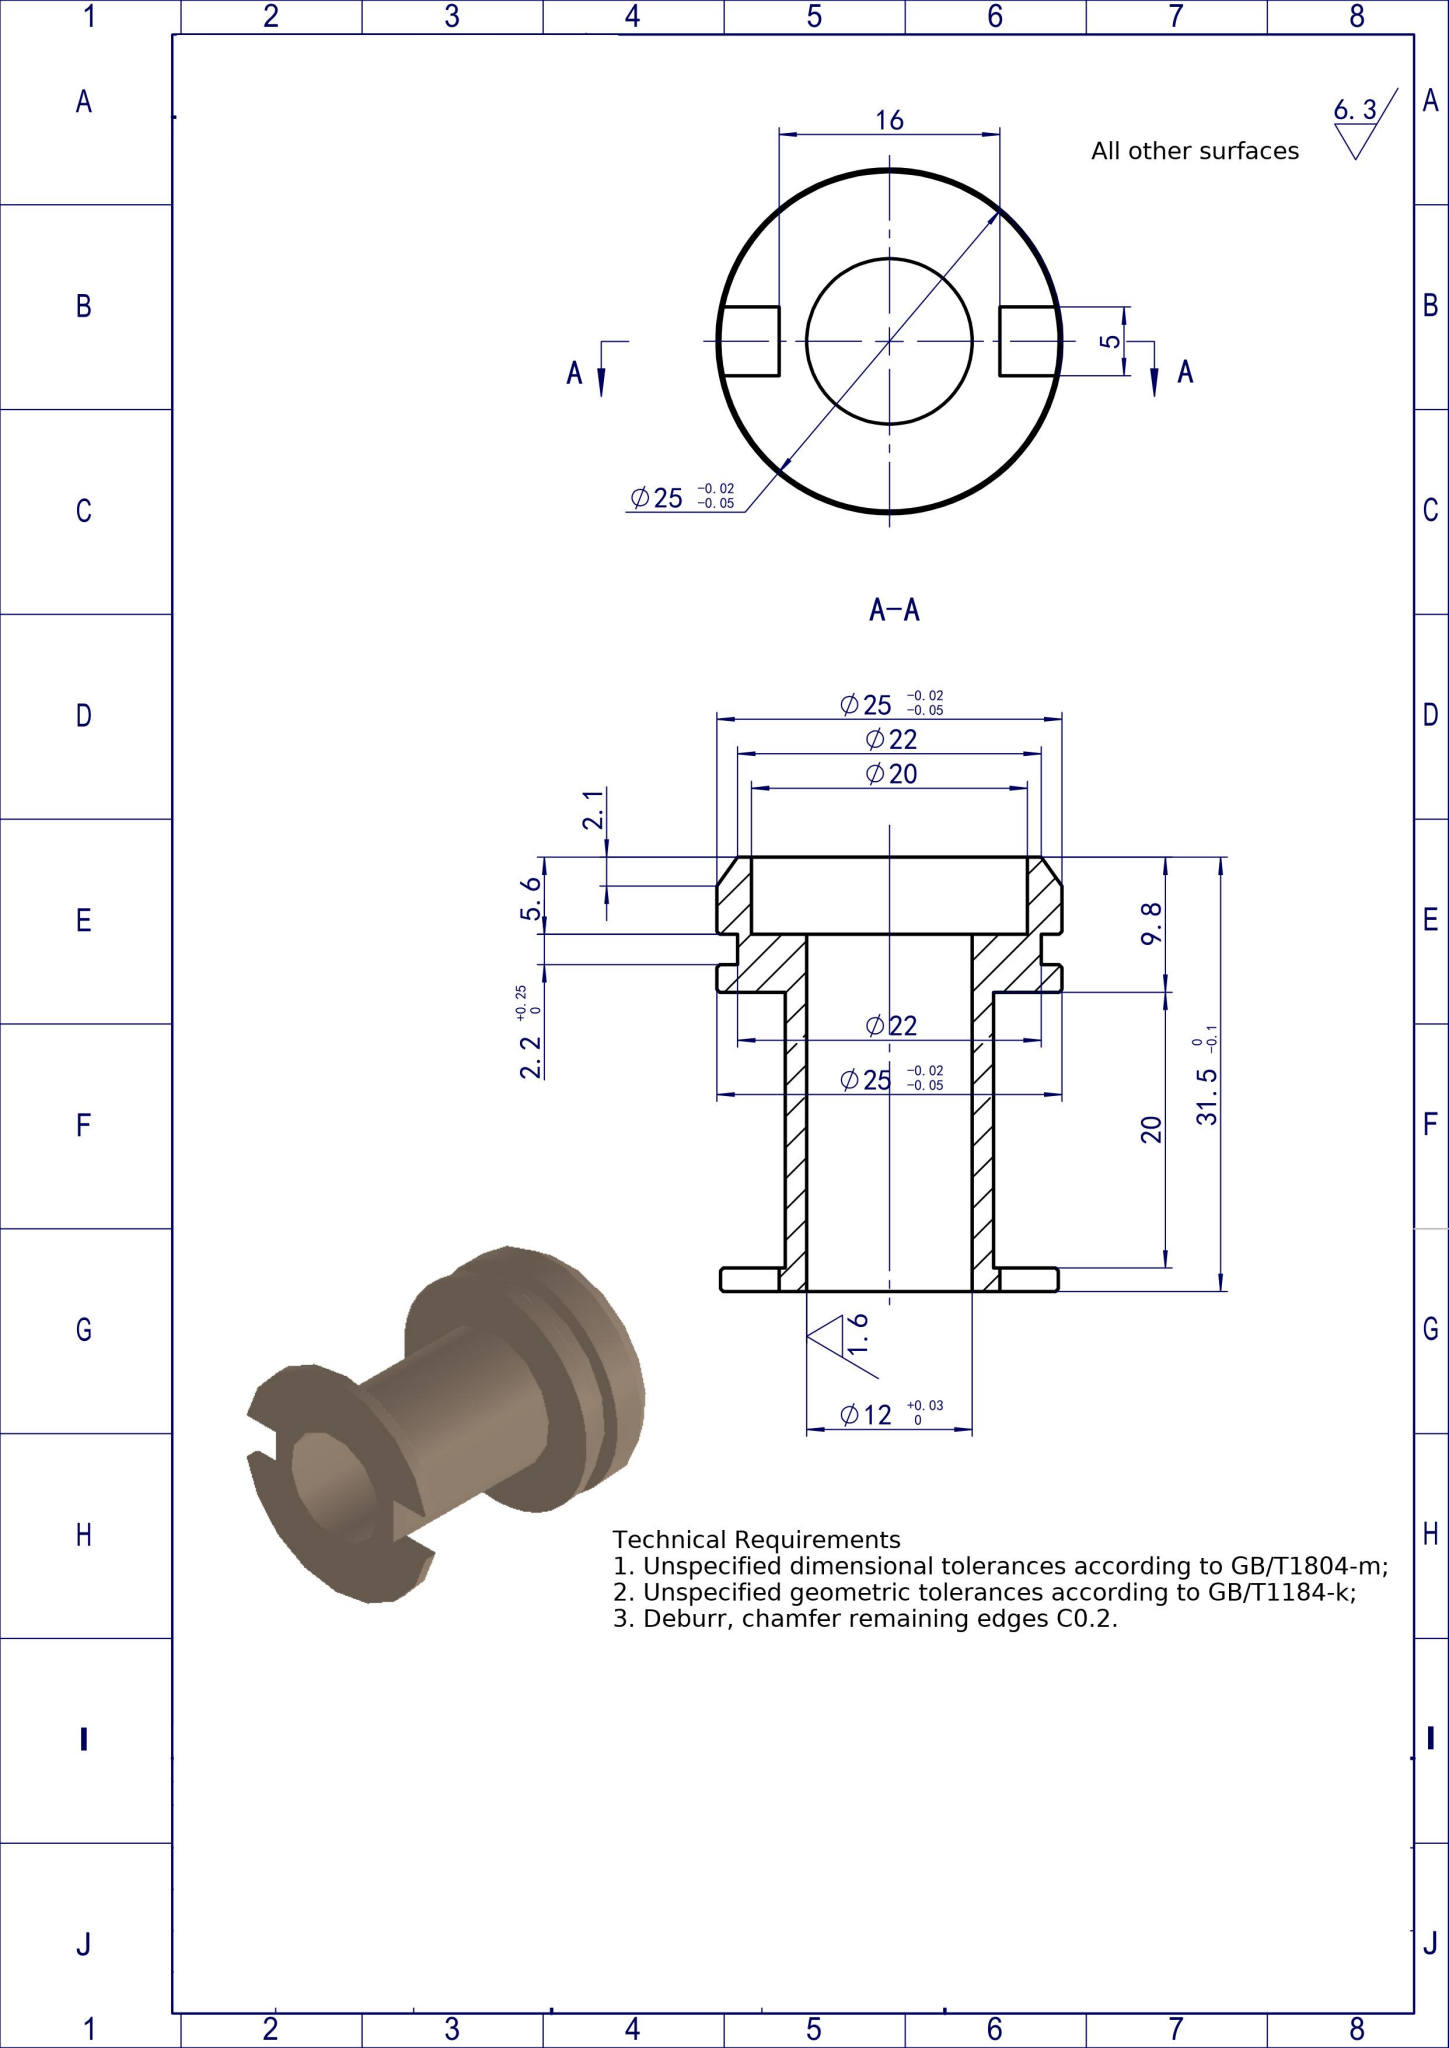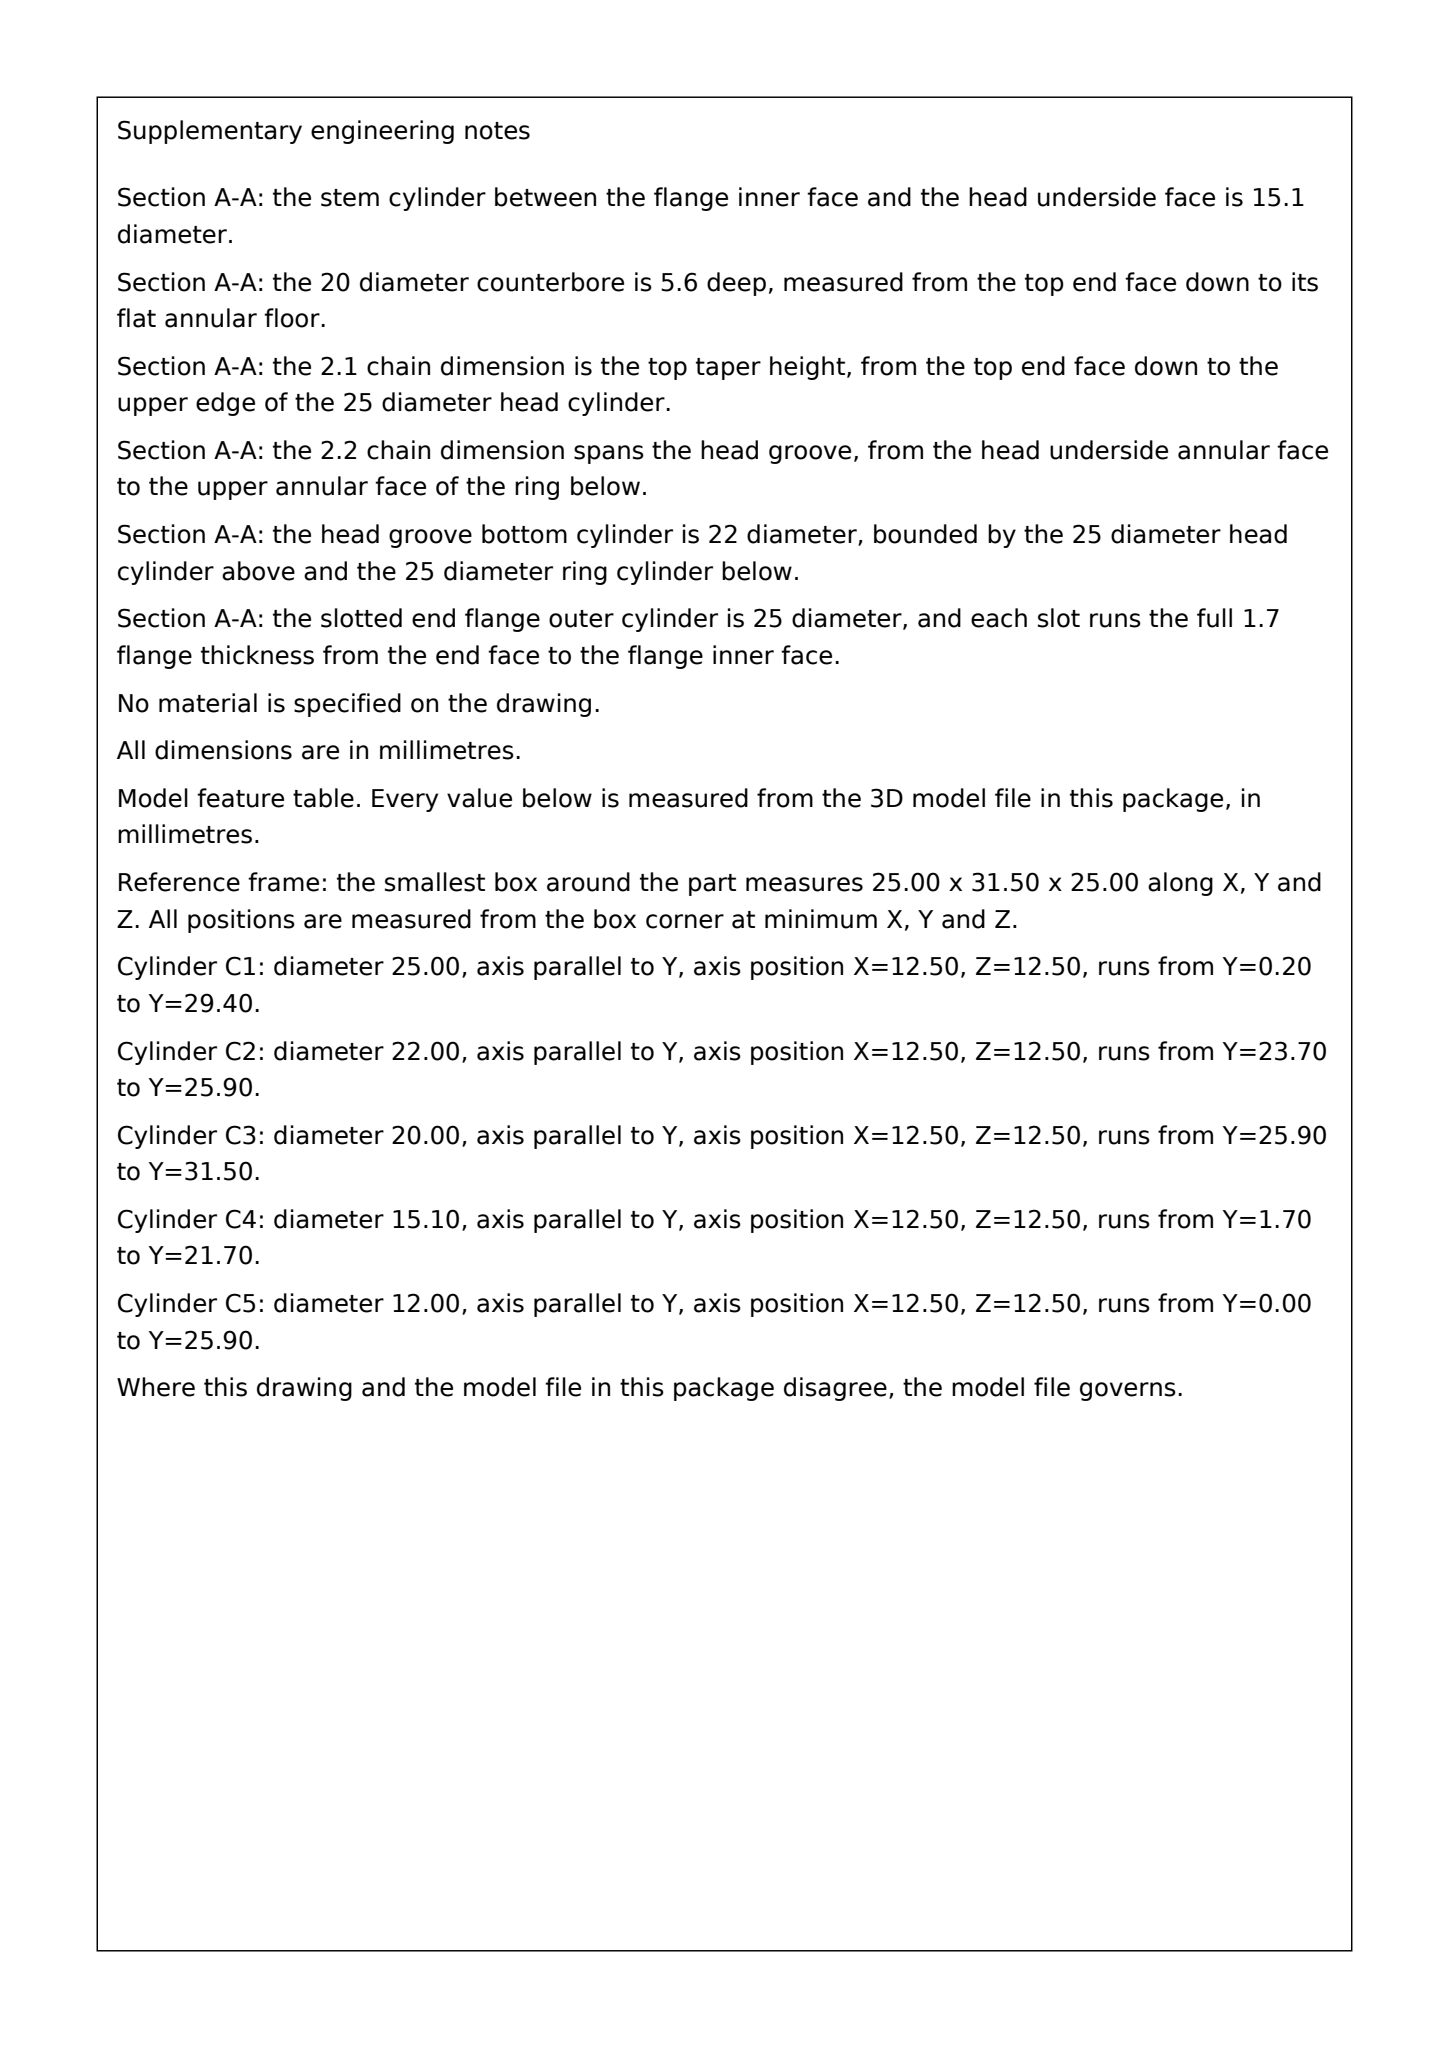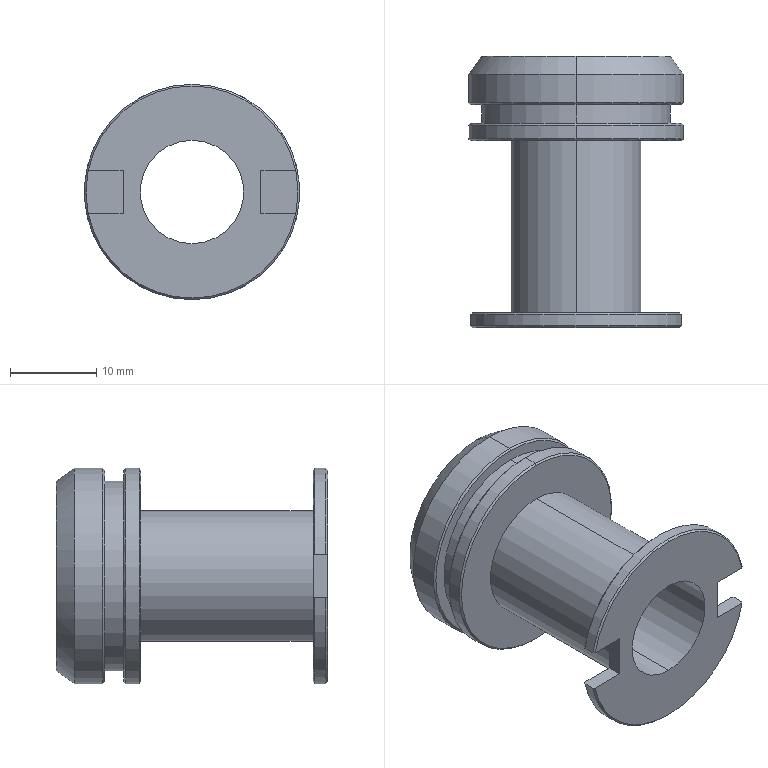Part | SolidWorks | mm | 1 solid | 42 faces | box 25 x 31.5 x 25 mm | volume 4093 mm3 | cylinder 15 | cone 14 | plane 13 | commonest cylinder face diameters 25 x7 20 x2 22 x2 15.1 x2 12 x2
Drawing notes:
2 SLOTS 5 WIDE x 16 ACROSS FLATS DP 5.6 FROM Ø25 FLANGE FACE | from the solid: Slot flats at x=4.5 & 20.5 (16 apart), walls z=10.0/15.0 (5 wide); slot floors = planes y=25.9 (2 off), i.e. 31.5-25.9=5.6 below flange face y=31.5
EXT GROOVE ON Ø25 FLANGE OD: 2.1 WIDE x Ø22 MINOR DIA | from the solid: Only sub-Ø25 external cyl in flange zone: Ø22 about axis y at [12.5,12.5], L=2.2, between Ø25 bands; drawing width 2.1
Ø25 BANDS 1.6 & 1.3 WIDE BTWN 5.6 AND 9.8 FROM FLANGE FACE | from the solid: Ø25 cyls L=1.6 and L=1.3 lie between planes y=21.7 and y=25.9, i.e. 9.8 and 5.6 below flange face y=31.5
FLANGE UNDERSIDE UNDERCUT: 71.1° INCL CONE FROM Ø25 AT 5.6 | from the solid: cones[71.1, ref_dia 25.0] x2 at flange underside, starts at Ø25 at plane y=25.9 = 5.6 from flange face y=31.5
Ø25 LANDS 3.3 & 1.6 WIDE: 2.1-5.4 AND 8.0-9.6 FROM TOP FACE | from the solid: Ø25 cyls L=3.3 (y 26.1-29.4) & L=1.6 (y 21.9-23.5); top face y=31.5; y-planes 21.7/23.7/25.9/31.5
RELIEF BTWN Ø25 LANDS: Ø22 x 2.2 WIDE; CHAMFER RUNOUT Ø24.6 | from the solid: Ø22 cyl L=2.2 between y-planes 23.7 and 25.9; 90° cones ref dia 24.6/25.0
Ø22 EXT GROOVE 2.2 WIDE, 5.6 FROM TOP FACE TO NEAR SIDE | from the solid: Ø22 cyl L=2.2 spans y 23.7-25.9; top face y=31.5 -> 31.5-25.9=5.6
ALL Ø25 LAND END EDGES C0.2 x 45° (TO Ø24.6) | from the solid: 90° included cones, ref dia 25.0 -> 24.6: 0.2 radial = 0.2 axial
build123d program:
from build123d import *

# Parameters (mm, degrees)
CHAMFER1_SIZE      = 0.2
CUT_EXTRUDE1_REACH = 38.121
SKETCH2_W          = 10
SKETCH2_H          = 5


with BuildPart() as part:
    # Sketch1 → Revolve1 (revolve)
    with BuildSketch(Plane.XY, mode=Mode.PRIVATE) as revolve1_sk:
        Polygon((6, 0), (12.5, 0), (12.5, 1.7), (7.55, 1.7), (7.55, 21.7), (12.5, 21.7), (12.5, 23.7), (11, 23.7), (11, 25.9), (12.5, 25.9), (12.5, 29.4), (11, 31.5), (10, 31.5), (10, 25.9), (6, 25.9), align=None)
    revolve(revolve1_sk.sketch.rotate(Axis((0, 0, 0), (0, 1, 0)), 90), axis=Axis((0, 0, 0), (0, 1, 0)))

    # Chamfer1
    chamfer1_edges = [part.edges().sort_by_distance(p)[0] for p in [
        (0, 25.9, 12.5),
        (0, 23.7, 12.5),
        (0, 21.7, 12.5),
        (0, 1.7, 12.5),
        (0, 0, 12.5),
    ]]
    chamfer(chamfer1_edges, length=CHAMFER1_SIZE)

    # Cut-Extrude1: up to this face of the body (flat: up to its plane)
    cut_extrude1_end = Plane(part.part.faces().sort_by_distance((0, 1.7, 11.952))[0])
    # Sketch2 → Cut-Extrude1 (cut, up to the picked face)
    with BuildSketch(Plane(origin=(0, 0, 0), x_dir=(-1, 0, 0), z_dir=(0, -1, 0)), mode=Mode.PRIVATE) as cut_extrude1_sk1:
        with Locations((-13, 0)):
            Rectangle(SKETCH2_W, SKETCH2_H)
    cut_extrude1_tool1 = split(extrude(cut_extrude1_sk1.sketch, amount=-CUT_EXTRUDE1_REACH, mode=Mode.PRIVATE), bisect_by=cut_extrude1_end, keep=Keep.BOTH, mode=Mode.PRIVATE)
    # Sketch2 → Cut-Extrude1 (cut, up to the picked face)
    with BuildSketch(Plane(origin=(0, 0, 0), x_dir=(-1, 0, 0), z_dir=(0, -1, 0)), mode=Mode.PRIVATE) as cut_extrude1_sk2:
        with Locations((13, 0)):
            Rectangle(SKETCH2_W, SKETCH2_H)
    cut_extrude1_tool2 = split(extrude(cut_extrude1_sk2.sketch, amount=-CUT_EXTRUDE1_REACH, mode=Mode.PRIVATE), bisect_by=cut_extrude1_end, keep=Keep.BOTH, mode=Mode.PRIVATE)
    add(cut_extrude1_tool1.solids().sort_by(Axis((13, 0, 0), (0, 1, 0)))[0], mode=Mode.SUBTRACT)
    add(cut_extrude1_tool2.solids().sort_by(Axis((-13, 0, 0), (0, 1, 0)))[0], mode=Mode.SUBTRACT)


solid = part.part